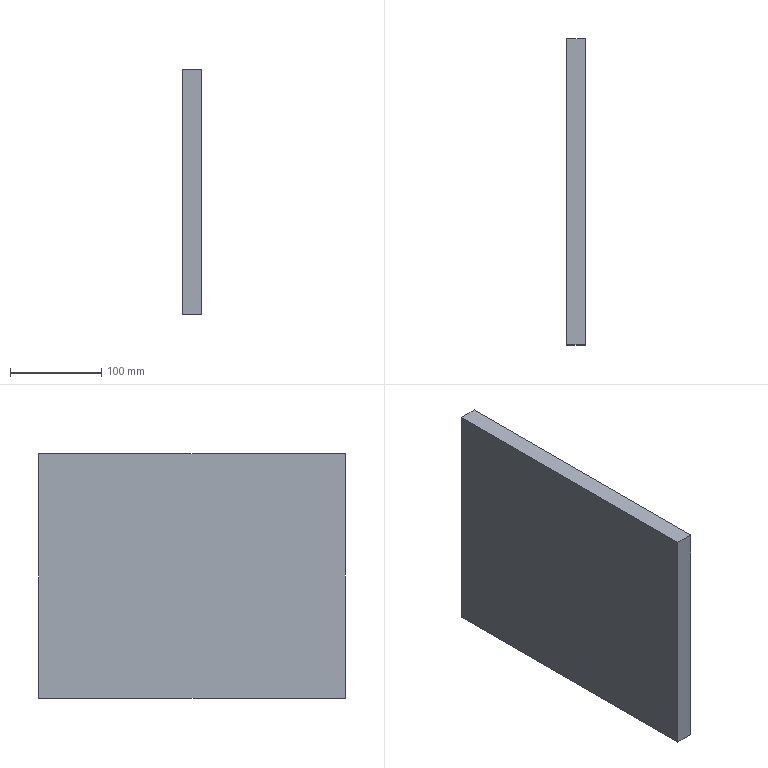Component | SolidWorks | HeatExchangePlate-1_PlateTwo-1 | 1 solid | 6 faces | box 20 x 334.74 x 267.35 mm | volume 1789855 mm3 | plane 6
build123d program:
from build123d import *

# Parameters (mm, degrees)
SKETCH1_W           = 267.35
SKETCH1_H           = 334.74
BOSS_EXTRUDE1_DEPTH = 20


with BuildPart() as part:
    # Sketch1 → Boss-Extrude1 (new body)
    with BuildSketch(Plane.XY):
        Rectangle(SKETCH1_W, SKETCH1_H)
    extrude(amount=BOSS_EXTRUDE1_DEPTH)


solid = part.part

# Placed as in the assembly
solid = solid.moved(Location((311.39, 652.58, 1.073), (0, 90, 0)))
STEP:
#1=CARTESIAN_POINT('',(13.047,19.103,5.305));
#2=VERTEX_POINT('',#1);
#3=CARTESIAN_POINT('',(13.047,32.281,5.305));
#4=VERTEX_POINT('',#3);
#5=CARTESIAN_POINT('',(13.047,32.281,5.305));
#6=DIRECTION('',(-0.,1.,0.));
#7=VECTOR('',#6,39.37);
#8=LINE('',#5,#7);
#9=EDGE_CURVE('',#2,#4,#8,.T.);
#10=ORIENTED_EDGE('',*,*,#9,.T.);
#11=CARTESIAN_POINT('',(12.259,32.281,5.305));
#12=VERTEX_POINT('',#11);
#13=CARTESIAN_POINT('',(12.259,32.281,5.305));
#14=DIRECTION('',(1.,0.,-0.));
#15=VECTOR('',#14,39.37);
#16=LINE('',#13,#15);
#17=EDGE_CURVE('',#12,#4,#16,.T.);
#18=ORIENTED_EDGE('',*,*,#17,.F.);
#19=CARTESIAN_POINT('',(12.259,19.103,5.305));
#20=VERTEX_POINT('',#19);
#21=CARTESIAN_POINT('',(12.259,32.281,5.305));
#22=DIRECTION('',(-0.,1.,0.));
#23=VECTOR('',#22,39.37);
#24=LINE('',#21,#23);
#25=EDGE_CURVE('',#20,#12,#24,.T.);
#26=ORIENTED_EDGE('',*,*,#25,.F.);
#27=CARTESIAN_POINT('',(12.259,19.103,5.305));
#28=DIRECTION('',(1.,0.,-0.));
#29=VECTOR('',#28,39.37);
#30=LINE('',#27,#29);
#31=EDGE_CURVE('',#20,#2,#30,.T.);
#32=ORIENTED_EDGE('',*,*,#31,.T.);
#33=EDGE_LOOP('',(#10,#18,#26,#32));
#34=FACE_OUTER_BOUND('',#33,.T.);
#35=CARTESIAN_POINT('',(12.259,32.281,5.305));
#36=DIRECTION('',(-0.,0.,-1.));
#37=DIRECTION('',(0.,-1.,-0.));
#38=AXIS2_PLACEMENT_3D('',#35,#36,#37);
#39=PLANE('',#38);
#40=ADVANCED_FACE('',(#34),#39,.F.);
#41=CARTESIAN_POINT('',(13.047,32.281,-5.221));
#42=VERTEX_POINT('',#41);
#43=CARTESIAN_POINT('',(13.047,32.281,-5.221));
#44=DIRECTION('',(-0.,0.,-1.));
#45=VECTOR('',#44,39.37);
#46=LINE('',#43,#45);
#47=EDGE_CURVE('',#4,#42,#46,.T.);
#48=ORIENTED_EDGE('',*,*,#47,.T.);
#49=CARTESIAN_POINT('',(12.259,32.281,-5.221));
#50=VERTEX_POINT('',#49);
#51=CARTESIAN_POINT('',(12.259,32.281,-5.221));
#52=DIRECTION('',(1.,0.,-0.));
#53=VECTOR('',#52,39.37);
#54=LINE('',#51,#53);
#55=EDGE_CURVE('',#50,#42,#54,.T.);
#56=ORIENTED_EDGE('',*,*,#55,.F.);
#57=CARTESIAN_POINT('',(12.259,32.281,-5.221));
#58=DIRECTION('',(-0.,0.,-1.));
#59=VECTOR('',#58,39.37);
#60=LINE('',#57,#59);
#61=EDGE_CURVE('',#12,#50,#60,.T.);
#62=ORIENTED_EDGE('',*,*,#61,.F.);
#63=ORIENTED_EDGE('',*,*,#17,.T.);
#64=EDGE_LOOP('',(#48,#56,#62,#63));
#65=FACE_OUTER_BOUND('',#64,.T.);
#66=CARTESIAN_POINT('',(12.259,32.281,-5.221));
#67=DIRECTION('',(0.,-1.,-0.));
#68=DIRECTION('',(1.,0.,-0.));
#69=AXIS2_PLACEMENT_3D('',#66,#67,#68);
#70=PLANE('',#69);
#71=ADVANCED_FACE('',(#65),#70,.F.);
#72=CARTESIAN_POINT('',(13.047,19.103,-5.221));
#73=VERTEX_POINT('',#72);
#74=CARTESIAN_POINT('',(13.047,32.281,-5.221));
#75=DIRECTION('',(0.,-1.,-0.));
#76=VECTOR('',#75,39.37);
#77=LINE('',#74,#76);
#78=EDGE_CURVE('',#42,#73,#77,.T.);
#79=ORIENTED_EDGE('',*,*,#78,.T.);
#80=CARTESIAN_POINT('',(12.259,19.103,-5.221));
#81=VERTEX_POINT('',#80);
#82=CARTESIAN_POINT('',(12.259,19.103,-5.221));
#83=DIRECTION('',(1.,0.,-0.));
#84=VECTOR('',#83,39.37);
#85=LINE('',#82,#84);
#86=EDGE_CURVE('',#81,#73,#85,.T.);
#87=ORIENTED_EDGE('',*,*,#86,.F.);
#88=CARTESIAN_POINT('',(12.259,32.281,-5.221));
#89=DIRECTION('',(0.,-1.,-0.));
#90=VECTOR('',#89,39.37);
#91=LINE('',#88,#90);
#92=EDGE_CURVE('',#50,#81,#91,.T.);
#93=ORIENTED_EDGE('',*,*,#92,.F.);
#94=ORIENTED_EDGE('',*,*,#55,.T.);
#95=EDGE_LOOP('',(#79,#87,#93,#94));
#96=FACE_OUTER_BOUND('',#95,.T.);
#97=CARTESIAN_POINT('',(12.259,32.281,-5.221));
#98=DIRECTION('',(0.,-0.,1.));
#99=DIRECTION('',(-0.,1.,0.));
#100=AXIS2_PLACEMENT_3D('',#97,#98,#99);
#101=PLANE('',#100);
#102=ADVANCED_FACE('',(#96),#101,.F.);
#103=CARTESIAN_POINT('',(13.047,19.103,-5.221));
#104=DIRECTION('',(0.,-0.,1.));
#105=VECTOR('',#104,39.37);
#106=LINE('',#103,#105);
#107=EDGE_CURVE('',#73,#2,#106,.T.);
#108=ORIENTED_EDGE('',*,*,#107,.T.);
#109=ORIENTED_EDGE('',*,*,#31,.F.);
#110=CARTESIAN_POINT('',(12.259,19.103,-5.221));
#111=DIRECTION('',(0.,-0.,1.));
#112=VECTOR('',#111,39.37);
#113=LINE('',#110,#112);
#114=EDGE_CURVE('',#81,#20,#113,.T.);
#115=ORIENTED_EDGE('',*,*,#114,.F.);
#116=ORIENTED_EDGE('',*,*,#86,.T.);
#117=EDGE_LOOP('',(#108,#109,#115,#116));
#118=FACE_OUTER_BOUND('',#117,.T.);
#119=CARTESIAN_POINT('',(12.259,19.103,-5.221));
#120=DIRECTION('',(-0.,1.,0.));
#121=DIRECTION('',(-1.,-0.,0.));
#122=AXIS2_PLACEMENT_3D('',#119,#120,#121);
#123=PLANE('',#122);
#124=ADVANCED_FACE('',(#118),#123,.F.);
#125=ORIENTED_EDGE('',*,*,#25,.T.);
#126=ORIENTED_EDGE('',*,*,#61,.T.);
#127=ORIENTED_EDGE('',*,*,#92,.T.);
#128=ORIENTED_EDGE('',*,*,#114,.T.);
#129=EDGE_LOOP('',(#125,#126,#127,#128));
#130=FACE_OUTER_BOUND('',#129,.T.);
#131=CARTESIAN_POINT('',(12.259,25.692,0.04226));
#132=DIRECTION('',(-1.,-0.,0.));
#133=DIRECTION('',(0.,-0.,1.));
#134=AXIS2_PLACEMENT_3D('',#131,#132,#133);
#135=PLANE('',#134);
#136=ADVANCED_FACE('',(#130),#135,.T.);
#137=ORIENTED_EDGE('',*,*,#9,.F.);
#138=ORIENTED_EDGE('',*,*,#107,.F.);
#139=ORIENTED_EDGE('',*,*,#78,.F.);
#140=ORIENTED_EDGE('',*,*,#47,.F.);
#141=EDGE_LOOP('',(#137,#138,#139,#140));
#142=FACE_OUTER_BOUND('',#141,.T.);
#143=CARTESIAN_POINT('',(13.047,25.692,0.04226));
#144=DIRECTION('',(-1.,-0.,0.));
#145=DIRECTION('',(0.,-0.,1.));
#146=AXIS2_PLACEMENT_3D('',#143,#144,#145);
#147=PLANE('',#146);
#148=ADVANCED_FACE('',(#142),#147,.F.);
#149=CLOSED_SHELL('',(#40,#71,#102,#124,#136,#148));
#150=MANIFOLD_SOLID_BREP('',#149);
#151=CARTESIAN_POINT('',(0.,0.,0.));
#152=DIRECTION('',(0.,0.,1.));
#153=DIRECTION('',(1.,0.,0.));
#154=AXIS2_PLACEMENT_3D('',#151,#152,#153);
#155=(LENGTH_UNIT()NAMED_UNIT(*)SI_UNIT($,.METRE.));
#156=LENGTH_MEASURE_WITH_UNIT(LENGTH_MEASURE(0.0254),#155);
#157=DIMENSIONAL_EXPONENTS(1.,0.,0.,0.,0.,0.,0.);
#158=(CONVERSION_BASED_UNIT('',#156)LENGTH_UNIT()NAMED_UNIT(#157));
#159=UNCERTAINTY_MEASURE_WITH_UNIT(LENGTH_MEASURE(0.00001),#158,'','');
#160=(NAMED_UNIT(*)PLANE_ANGLE_UNIT()SI_UNIT($,.RADIAN.));
#161=(NAMED_UNIT(*)SI_UNIT($,.STERADIAN.)SOLID_ANGLE_UNIT());
#162=(GEOMETRIC_REPRESENTATION_CONTEXT(3)GLOBAL_UNCERTAINTY_ASSIGNED_CONTEXT((#159))GLOBAL_UNIT_ASSIGNED_CONTEXT((#158,#160,#161))REPRESENTATION_CONTEXT('',''));
#163=ADVANCED_BREP_SHAPE_REPRESENTATION('',(#150,#154),#162);
#164=COLOUR_RGB('',0.7922,0.8196,0.9333);
#165=FILL_AREA_STYLE_COLOUR('',#164);
#166=FILL_AREA_STYLE('',(#165));
#167=SURFACE_STYLE_FILL_AREA(#166);
#168=SURFACE_SIDE_STYLE('',(#167));
#169=SURFACE_STYLE_USAGE(.BOTH.,#168);
#170=PRESENTATION_STYLE_ASSIGNMENT((#169));
#171=STYLED_ITEM('',(#170),#150);
#172=(LENGTH_UNIT()NAMED_UNIT(*)SI_UNIT($,.METRE.));
#173=LENGTH_MEASURE_WITH_UNIT(LENGTH_MEASURE(0.0254),#172);
#174=DIMENSIONAL_EXPONENTS(1.,0.,0.,0.,0.,0.,0.);
#175=(CONVERSION_BASED_UNIT('',#173)LENGTH_UNIT()NAMED_UNIT(#174));
#176=UNCERTAINTY_MEASURE_WITH_UNIT(LENGTH_MEASURE(0.00001),#175,'','');
#177=(NAMED_UNIT(*)PLANE_ANGLE_UNIT()SI_UNIT($,.RADIAN.));
#178=(NAMED_UNIT(*)SI_UNIT($,.STERADIAN.)SOLID_ANGLE_UNIT());
#179=(GEOMETRIC_REPRESENTATION_CONTEXT(3)GLOBAL_UNCERTAINTY_ASSIGNED_CONTEXT((#176))GLOBAL_UNIT_ASSIGNED_CONTEXT((#175,#177,#178))REPRESENTATION_CONTEXT('',''));
#180=MECHANICAL_DESIGN_GEOMETRIC_PRESENTATION_REPRESENTATION('',(#171),#179);
#181=PRESENTATION_LAYER_ASSIGNMENT('','',(#171));